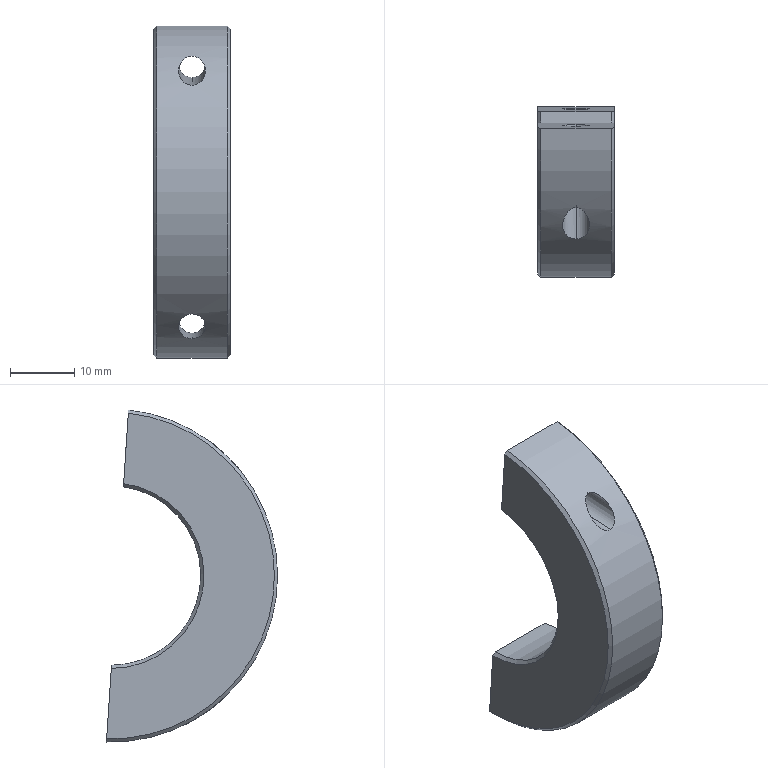Component | SolidWorks | TC020.05-08-1 | 1 solid | 14 faces | box 12 x 26.73 x 51.86 mm | volume 8299 mm3 | cylinder 6 | plane 4 | cone 4 | commonest cylinder face diameters 4.2 x4 28 x1 52 x1 | material Q235A
build123d program:
from build123d import *

# Parameters (mm, degrees)
SKETCH1_W          = 12
SKETCH1_H          = 12
SKETCH2_W          = 52
SKETCH2_H          = 2
CUT_EXTRUDE1_DEPTH = 39.678
M5_TAPPED_HOLE1_D  = 4.2
CHAMFER1_SIZE      = 0.5


with BuildPart() as part:
    # Sketch1 → Revolve1 (revolve)
    with BuildSketch(Plane.XY, mode=Mode.PRIVATE) as revolve1_sk:
        with Locations((0, 20)):
            Rectangle(SKETCH1_W, SKETCH1_H)
    revolve(revolve1_sk.sketch.rotate(Axis((0, 0, 0), (1, 0, 0)), 90), axis=Axis((0, 0, 0), (1, 0, 0)))

    # Sketch2 → Cut-Extrude1 (cut, through all)
    with BuildSketch(Plane(origin=(6, 0, 0), x_dir=(0, 0, -1), z_dir=(1, 0, 0))):
        Rectangle(SKETCH2_W, SKETCH2_H)
    extrude(amount=-CUT_EXTRUDE1_DEPTH, mode=Mode.SUBTRACT)


with BuildPart() as cut_extrude1_kept_piece:
    # of the separate pieces the step leaves, the one the design keeps (cut_extrude1_pieces_kept)
    add(part.part.solids().sort_by_distance((-6, 1, -13.964))[0])

    # M5 Tapped Hole1 (through all)
    with Locations(Plane.XZ.offset(-1)):
        with Locations((0, 20), (0, -20)):
            Hole(M5_TAPPED_HOLE1_D / 2)

    # Chamfer1
    chamfer1_edges = [cut_extrude1_kept_piece.edges().sort_by_distance(p)[0] for p in [
        (6, 26, 0),
        (-6, 26, 0),
        (-6, 14, 0),
        (6, 14, 0),
    ]]
    chamfer(chamfer1_edges, length=CHAMFER1_SIZE)


solid = cut_extrude1_kept_piece.part

# Placed as in the assembly
solid = solid.moved(Location((239.493, 30, 0), (3.804, 0, -180)))
STEP:
#1=COLOUR_RGB('',0.7922,0.8196,0.9333);
#2=FILL_AREA_STYLE_COLOUR('',#1);
#3=FILL_AREA_STYLE('',(#2));
#4=SURFACE_STYLE_FILL_AREA(#3);
#5=SURFACE_SIDE_STYLE('',(#4));
#6=SURFACE_STYLE_USAGE(.BOTH.,#5);
#7=PRESENTATION_STYLE_ASSIGNMENT((#6));
#8=CARTESIAN_POINT('',(9.429,0.7008,-0.9039));
#9=VERTEX_POINT('',#8);
#10=CARTESIAN_POINT('',(9.429,0.4871,-0.7524));
#11=VERTEX_POINT('',#10);
#12=CARTESIAN_POINT('',(9.429,0.7008,-0.9039));
#13=CARTESIAN_POINT('',(9.425,0.7008,-0.9039));
#14=CARTESIAN_POINT('',(9.422,0.7004,-0.9037));
#15=CARTESIAN_POINT('',(9.415,0.6989,-0.9029));
#16=CARTESIAN_POINT('',(9.411,0.6978,-0.9023));
#17=CARTESIAN_POINT('',(9.402,0.6937,-0.9001));
#18=CARTESIAN_POINT('',(9.396,0.6899,-0.8981));
#19=CARTESIAN_POINT('',(9.386,0.6813,-0.8933));
#20=CARTESIAN_POINT('',(9.381,0.6765,-0.8906));
#21=CARTESIAN_POINT('',(9.373,0.6663,-0.8848));
#22=CARTESIAN_POINT('',(9.37,0.6611,-0.8817));
#23=CARTESIAN_POINT('',(9.36,0.6448,-0.872));
#24=CARTESIAN_POINT('',(9.355,0.6333,-0.8648));
#25=CARTESIAN_POINT('',(9.349,0.6103,-0.8498));
#26=CARTESIAN_POINT('',(9.347,0.5988,-0.842));
#27=CARTESIAN_POINT('',(9.346,0.5816,-0.8297));
#28=CARTESIAN_POINT('',(9.346,0.5758,-0.8255));
#29=CARTESIAN_POINT('',(9.347,0.5645,-0.8171));
#30=CARTESIAN_POINT('',(9.348,0.5589,-0.8129));
#31=CARTESIAN_POINT('',(9.352,0.5425,-0.8001));
#32=CARTESIAN_POINT('',(9.356,0.5318,-0.7915));
#33=CARTESIAN_POINT('',(9.369,0.5126,-0.7753));
#34=CARTESIAN_POINT('',(9.378,0.5039,-0.7676));
#35=CARTESIAN_POINT('',(9.395,0.4942,-0.759));
#36=CARTESIAN_POINT('',(9.401,0.4916,-0.7566));
#37=CARTESIAN_POINT('',(9.411,0.4889,-0.7541));
#38=CARTESIAN_POINT('',(9.415,0.4883,-0.7535));
#39=CARTESIAN_POINT('',(9.422,0.4873,-0.7526));
#40=CARTESIAN_POINT('',(9.425,0.4871,-0.7524));
#41=CARTESIAN_POINT('',(9.429,0.4871,-0.7524));
#42=B_SPLINE_CURVE_WITH_KNOTS('',3,(#12,#13,#14,#15,#16,#17,#18,#19,#20,#21,#22,#23,#24,#25,#26,#27,#28,#29,#30,#31,#32,#33,#34,#35,#36,#37,#38,#39,#40,#41),.UNSPECIFIED.,.F.,.F.,(4,2,2,2,2,2,2,2,2,2,2,2,2,2,4),(0.008626,0.008896,0.009166,0.009706,0.01025,0.01079,0.01187,0.01295,0.01349,0.01403,0.01511,0.01619,0.01673,0.017,0.01727),.UNSPECIFIED.);
#43=EDGE_CURVE('',#9,#11,#42,.T.);
#44=ORIENTED_EDGE('',*,*,#43,.F.);
#45=CARTESIAN_POINT('',(9.429,1.2,-0.8708));
#46=VERTEX_POINT('',#45);
#47=CARTESIAN_POINT('',(9.429,1.2,-0.8708));
#48=DIRECTION('',(0.,0.9978,0.06635));
#49=VECTOR('',#48,39.37);
#50=LINE('',#47,#49);
#51=EDGE_CURVE('',#9,#46,#50,.T.);
#52=ORIENTED_EDGE('',*,*,#51,.T.);
#53=CARTESIAN_POINT('',(9.429,1.189,-0.7058));
#54=VERTEX_POINT('',#53);
#55=CARTESIAN_POINT('',(9.429,1.194,-0.7883));
#56=DIRECTION('',(0.,0.9978,0.06635));
#57=DIRECTION('',(0.,-0.06635,0.9978));
#58=AXIS2_PLACEMENT_3D('',#55,#56,#57);
#59=CIRCLE('',#58,0.08268);
#60=EDGE_CURVE('',#46,#54,#59,.T.);
#61=ORIENTED_EDGE('',*,*,#60,.T.);
#62=CARTESIAN_POINT('',(9.429,1.189,-0.7058));
#63=DIRECTION('',(0.,0.9978,0.06635));
#64=VECTOR('',#63,39.37);
#65=LINE('',#62,#64);
#66=EDGE_CURVE('',#11,#54,#65,.T.);
#67=ORIENTED_EDGE('',*,*,#66,.F.);
#68=EDGE_LOOP('',(#44,#52,#61,#67));
#69=FACE_OUTER_BOUND('',#68,.T.);
#70=CARTESIAN_POINT('',(9.429,1.194,-0.7883));
#71=DIRECTION('',(0.,0.9978,0.06635));
#72=DIRECTION('',(0.,-0.06635,0.9978));
#73=AXIS2_PLACEMENT_3D('',#70,#71,#72);
#74=CYLINDRICAL_SURFACE('',#73,0.08268);
#75=ADVANCED_FACE('',(#69),#74,.F.);
#76=CARTESIAN_POINT('',(9.429,0.3936,0.6539));
#77=VERTEX_POINT('',#76);
#78=CARTESIAN_POINT('',(9.429,0.5853,0.8324));
#79=VERTEX_POINT('',#78);
#80=CARTESIAN_POINT('',(9.429,0.3936,0.6539));
#81=CARTESIAN_POINT('',(9.422,0.3936,0.6539));
#82=CARTESIAN_POINT('',(9.415,0.3944,0.6549));
#83=CARTESIAN_POINT('',(9.401,0.3975,0.6586));
#84=CARTESIAN_POINT('',(9.395,0.3998,0.6613));
#85=CARTESIAN_POINT('',(9.384,0.4054,0.6679));
#86=CARTESIAN_POINT('',(9.379,0.4087,0.6718));
#87=CARTESIAN_POINT('',(9.37,0.416,0.6801));
#88=CARTESIAN_POINT('',(9.366,0.4201,0.6846));
#89=CARTESIAN_POINT('',(9.356,0.4328,0.6986));
#90=CARTESIAN_POINT('',(9.352,0.4421,0.7084));
#91=CARTESIAN_POINT('',(9.347,0.4617,0.7284));
#92=CARTESIAN_POINT('',(9.346,0.4718,0.7382));
#93=CARTESIAN_POINT('',(9.347,0.4923,0.7574));
#94=CARTESIAN_POINT('',(9.349,0.5029,0.7669));
#95=CARTESIAN_POINT('',(9.356,0.5236,0.7847));
#96=CARTESIAN_POINT('',(9.36,0.5339,0.7932));
#97=CARTESIAN_POINT('',(9.37,0.5489,0.8051));
#98=CARTESIAN_POINT('',(9.373,0.5538,0.8089));
#99=CARTESIAN_POINT('',(9.381,0.563,0.816));
#100=CARTESIAN_POINT('',(9.386,0.5675,0.8193));
#101=CARTESIAN_POINT('',(9.396,0.5753,0.8251));
#102=CARTESIAN_POINT('',(9.402,0.5788,0.8277));
#103=CARTESIAN_POINT('',(9.415,0.5838,0.8313));
#104=CARTESIAN_POINT('',(9.422,0.5853,0.8324));
#105=CARTESIAN_POINT('',(9.429,0.5853,0.8324));
#106=B_SPLINE_CURVE_WITH_KNOTS('',3,(#80,#81,#82,#83,#84,#85,#86,#87,#88,#89,#90,#91,#92,#93,#94,#95,#96,#97,#98,#99,#100,#101,#102,#103,#104,#105),.UNSPECIFIED.,.F.,.F.,(4,2,2,2,2,2,2,2,2,2,2,2,4),(0.008659,0.0092,0.009741,0.01028,0.01082,0.0119,0.01299,0.01407,0.01515,0.01569,0.01623,0.01677,0.01731),.UNSPECIFIED.);
#107=EDGE_CURVE('',#77,#79,#106,.T.);
#108=ORIENTED_EDGE('',*,*,#107,.F.);
#109=CARTESIAN_POINT('',(9.429,1.095,0.7006));
#110=VERTEX_POINT('',#109);
#111=CARTESIAN_POINT('',(9.429,1.095,0.7006));
#112=DIRECTION('',(0.,0.9978,0.06635));
#113=VECTOR('',#112,39.37);
#114=LINE('',#111,#113);
#115=EDGE_CURVE('',#77,#110,#114,.T.);
#116=ORIENTED_EDGE('',*,*,#115,.T.);
#117=CARTESIAN_POINT('',(9.429,1.084,0.8655));
#118=VERTEX_POINT('',#117);
#119=CARTESIAN_POINT('',(9.429,1.09,0.7831));
#120=DIRECTION('',(0.,0.9978,0.06635));
#121=DIRECTION('',(0.,-0.06635,0.9978));
#122=AXIS2_PLACEMENT_3D('',#119,#120,#121);
#123=CIRCLE('',#122,0.08268);
#124=EDGE_CURVE('',#110,#118,#123,.T.);
#125=ORIENTED_EDGE('',*,*,#124,.T.);
#126=CARTESIAN_POINT('',(9.429,1.084,0.8655));
#127=DIRECTION('',(0.,0.9978,0.06635));
#128=VECTOR('',#127,39.37);
#129=LINE('',#126,#128);
#130=EDGE_CURVE('',#79,#118,#129,.T.);
#131=ORIENTED_EDGE('',*,*,#130,.F.);
#132=EDGE_LOOP('',(#108,#116,#125,#131));
#133=FACE_OUTER_BOUND('',#132,.T.);
#134=CARTESIAN_POINT('',(9.429,1.09,0.7831));
#135=DIRECTION('',(0.,0.9978,0.06635));
#136=DIRECTION('',(0.,-0.06635,0.9978));
#137=AXIS2_PLACEMENT_3D('',#134,#135,#136);
#138=CYLINDRICAL_SURFACE('',#137,0.08268);
#139=ADVANCED_FACE('',(#133),#138,.F.);
#140=CARTESIAN_POINT('',(9.645,1.178,-0.5512));
#141=VERTEX_POINT('',#140);
#142=CARTESIAN_POINT('',(9.212,1.178,-0.5512));
#143=VERTEX_POINT('',#142);
#144=CARTESIAN_POINT('',(9.429,1.178,-0.5512));
#145=DIRECTION('',(-1.,0.,0.));
#146=VECTOR('',#145,39.37);
#147=LINE('',#144,#146);
#148=EDGE_CURVE('',#141,#143,#147,.T.);
#149=ORIENTED_EDGE('',*,*,#148,.T.);
#150=CARTESIAN_POINT('',(9.212,1.105,0.5459));
#151=VERTEX_POINT('',#150);
#152=CARTESIAN_POINT('',(9.212,1.181,0.));
#153=DIRECTION('',(-1.,0.,0.));
#154=DIRECTION('',(0.,-0.06635,0.9978));
#155=AXIS2_PLACEMENT_3D('',#152,#153,#154);
#156=CIRCLE('',#155,0.5512);
#157=EDGE_CURVE('',#143,#151,#156,.T.);
#158=ORIENTED_EDGE('',*,*,#157,.T.);
#159=CARTESIAN_POINT('',(9.645,1.105,0.5459));
#160=VERTEX_POINT('',#159);
#161=CARTESIAN_POINT('',(9.429,1.105,0.5459));
#162=DIRECTION('',(1.,0.,0.));
#163=VECTOR('',#162,39.37);
#164=LINE('',#161,#163);
#165=EDGE_CURVE('',#151,#160,#164,.T.);
#166=ORIENTED_EDGE('',*,*,#165,.T.);
#167=CARTESIAN_POINT('',(9.645,1.181,0.));
#168=DIRECTION('',(1.,0.,0.));
#169=DIRECTION('',(0.,0.06635,-0.9978));
#170=AXIS2_PLACEMENT_3D('',#167,#168,#169);
#171=CIRCLE('',#170,0.5512);
#172=EDGE_CURVE('',#160,#141,#171,.T.);
#173=ORIENTED_EDGE('',*,*,#172,.T.);
#174=EDGE_LOOP('',(#149,#158,#166,#173));
#175=FACE_OUTER_BOUND('',#174,.T.);
#176=CARTESIAN_POINT('',(9.429,1.181,0.));
#177=DIRECTION('',(-1.,0.,0.));
#178=DIRECTION('',(0.,0.06635,-0.9978));
#179=AXIS2_PLACEMENT_3D('',#176,#177,#178);
#180=CYLINDRICAL_SURFACE('',#179,0.5512);
#181=ADVANCED_FACE('',(#175),#180,.F.);
#182=CARTESIAN_POINT('',(9.665,1.18,-0.5709));
#183=VERTEX_POINT('',#182);
#184=CARTESIAN_POINT('',(9.665,1.208,-1.004));
#185=VERTEX_POINT('',#184);
#186=CARTESIAN_POINT('',(9.665,1.21,-1.024));
#187=DIRECTION('',(0.,0.06635,-0.9978));
#188=VECTOR('',#187,39.37);
#189=LINE('',#186,#188);
#190=EDGE_CURVE('',#183,#185,#189,.T.);
#191=ORIENTED_EDGE('',*,*,#190,.F.);
#192=CARTESIAN_POINT('',(9.665,1.104,0.5656));
#193=VERTEX_POINT('',#192);
#194=CARTESIAN_POINT('',(9.665,1.181,0.));
#195=DIRECTION('',(-1.,0.,0.));
#196=DIRECTION('',(0.,0.06635,-0.9978));
#197=AXIS2_PLACEMENT_3D('',#194,#195,#196);
#198=CIRCLE('',#197,0.5709);
#199=EDGE_CURVE('',#183,#193,#198,.T.);
#200=ORIENTED_EDGE('',*,*,#199,.T.);
#201=CARTESIAN_POINT('',(9.665,1.075,0.9983));
#202=VERTEX_POINT('',#201);
#203=CARTESIAN_POINT('',(9.665,1.21,-1.024));
#204=DIRECTION('',(0.,0.06635,-0.9978));
#205=VECTOR('',#204,39.37);
#206=LINE('',#203,#205);
#207=EDGE_CURVE('',#202,#193,#206,.T.);
#208=ORIENTED_EDGE('',*,*,#207,.F.);
#209=CARTESIAN_POINT('',(9.665,1.181,0.));
#210=DIRECTION('',(1.,0.,0.));
#211=DIRECTION('',(0.,0.06635,-0.9978));
#212=AXIS2_PLACEMENT_3D('',#209,#210,#211);
#213=CIRCLE('',#212,1.004);
#214=EDGE_CURVE('',#202,#185,#213,.T.);
#215=ORIENTED_EDGE('',*,*,#214,.T.);
#216=EDGE_LOOP('',(#191,#200,#208,#215));
#217=FACE_OUTER_BOUND('',#216,.T.);
#218=CARTESIAN_POINT('',(9.665,0.6311,-0.03657));
#219=DIRECTION('',(-1.,0.,0.));
#220=DIRECTION('',(0.,0.06635,-0.9978));
#221=AXIS2_PLACEMENT_3D('',#218,#219,#220);
#222=PLANE('',#221);
#223=ADVANCED_FACE('',(#217),#222,.F.);
#224=CARTESIAN_POINT('',(9.429,0.4871,-0.7524));
#225=CARTESIAN_POINT('',(9.436,0.4871,-0.7524));
#226=CARTESIAN_POINT('',(9.443,0.488,-0.7533));
#227=CARTESIAN_POINT('',(9.456,0.4916,-0.7566));
#228=CARTESIAN_POINT('',(9.463,0.4942,-0.7589));
#229=CARTESIAN_POINT('',(9.474,0.5007,-0.7647));
#230=CARTESIAN_POINT('',(9.479,0.5044,-0.7681));
#231=CARTESIAN_POINT('',(9.488,0.5128,-0.7753));
#232=CARTESIAN_POINT('',(9.492,0.5174,-0.7793));
#233=CARTESIAN_POINT('',(9.498,0.527,-0.7874));
#234=CARTESIAN_POINT('',(9.501,0.532,-0.7916));
#235=CARTESIAN_POINT('',(9.505,0.5425,-0.8));
#236=CARTESIAN_POINT('',(9.507,0.5479,-0.8043));
#237=CARTESIAN_POINT('',(9.511,0.5644,-0.8171));
#238=CARTESIAN_POINT('',(9.512,0.5757,-0.8255));
#239=CARTESIAN_POINT('',(9.511,0.5987,-0.8419));
#240=CARTESIAN_POINT('',(9.509,0.6104,-0.8499));
#241=CARTESIAN_POINT('',(9.502,0.6333,-0.8648));
#242=CARTESIAN_POINT('',(9.497,0.6448,-0.872));
#243=CARTESIAN_POINT('',(9.488,0.6611,-0.8817));
#244=CARTESIAN_POINT('',(9.485,0.6664,-0.8848));
#245=CARTESIAN_POINT('',(9.476,0.6765,-0.8906));
#246=CARTESIAN_POINT('',(9.472,0.6813,-0.8933));
#247=CARTESIAN_POINT('',(9.462,0.6899,-0.8981));
#248=CARTESIAN_POINT('',(9.456,0.6937,-0.9001));
#249=CARTESIAN_POINT('',(9.443,0.6992,-0.9031));
#250=CARTESIAN_POINT('',(9.436,0.7008,-0.9039));
#251=CARTESIAN_POINT('',(9.429,0.7008,-0.9039));
#252=B_SPLINE_CURVE_WITH_KNOTS('',3,(#224,#225,#226,#227,#228,#229,#230,#231,#232,#233,#234,#235,#236,#237,#238,#239,#240,#241,#242,#243,#244,#245,#246,#247,#248,#249,#250,#251),.UNSPECIFIED.,.F.,.F.,(4,2,2,2,2,2,2,2,2,2,2,2,2,4),(0.,0.0005391,0.001078,0.001617,0.002156,0.002696,0.003235,0.004313,0.005391,0.006469,0.007008,0.007547,0.008087,0.008626),.UNSPECIFIED.);
#253=EDGE_CURVE('',#11,#9,#252,.T.);
#254=ORIENTED_EDGE('',*,*,#253,.T.);
#255=ORIENTED_EDGE('',*,*,#43,.T.);
#256=EDGE_LOOP('',(#254,#255));
#257=FACE_BOUND('',#256,.T.);
#258=CARTESIAN_POINT('',(9.429,0.5853,0.8324));
#259=CARTESIAN_POINT('',(9.432,0.5853,0.8324));
#260=CARTESIAN_POINT('',(9.436,0.585,0.8321));
#261=CARTESIAN_POINT('',(9.443,0.5836,0.8311));
#262=CARTESIAN_POINT('',(9.446,0.5826,0.8304));
#263=CARTESIAN_POINT('',(9.456,0.5788,0.8277));
#264=CARTESIAN_POINT('',(9.462,0.5753,0.8251));
#265=CARTESIAN_POINT('',(9.477,0.5635,0.8164));
#266=CARTESIAN_POINT('',(9.485,0.5538,0.809));
#267=CARTESIAN_POINT('',(9.494,0.539,0.7972));
#268=CARTESIAN_POINT('',(9.497,0.5339,0.7931));
#269=CARTESIAN_POINT('',(9.502,0.5237,0.7846));
#270=CARTESIAN_POINT('',(9.504,0.5184,0.7802));
#271=CARTESIAN_POINT('',(9.509,0.5028,0.7667));
#272=CARTESIAN_POINT('',(9.511,0.4924,0.7575));
#273=CARTESIAN_POINT('',(9.512,0.4719,0.7382));
#274=CARTESIAN_POINT('',(9.511,0.4616,0.7282));
#275=CARTESIAN_POINT('',(9.507,0.447,0.7134));
#276=CARTESIAN_POINT('',(9.505,0.4423,0.7085));
#277=CARTESIAN_POINT('',(9.501,0.433,0.6987));
#278=CARTESIAN_POINT('',(9.498,0.4285,0.6938));
#279=CARTESIAN_POINT('',(9.489,0.4158,0.6799));
#280=CARTESIAN_POINT('',(9.48,0.4082,0.6712));
#281=CARTESIAN_POINT('',(9.463,0.3998,0.6613));
#282=CARTESIAN_POINT('',(9.456,0.3975,0.6586));
#283=CARTESIAN_POINT('',(9.446,0.3952,0.6558));
#284=CARTESIAN_POINT('',(9.443,0.3946,0.6551));
#285=CARTESIAN_POINT('',(9.436,0.3938,0.6542));
#286=CARTESIAN_POINT('',(9.432,0.3936,0.6539));
#287=CARTESIAN_POINT('',(9.429,0.3936,0.6539));
#288=B_SPLINE_CURVE_WITH_KNOTS('',3,(#258,#259,#260,#261,#262,#263,#264,#265,#266,#267,#268,#269,#270,#271,#272,#273,#274,#275,#276,#277,#278,#279,#280,#281,#282,#283,#284,#285,#286,#287),.UNSPECIFIED.,.F.,.F.,(4,2,2,2,2,2,2,2,2,2,2,2,2,2,4),(0.,0.0002706,0.0005412,0.001082,0.002165,0.002706,0.003247,0.004329,0.005412,0.005953,0.006494,0.007577,0.008118,0.008388,0.008659),.UNSPECIFIED.);
#289=EDGE_CURVE('',#79,#77,#288,.T.);
#290=ORIENTED_EDGE('',*,*,#289,.T.);
#291=ORIENTED_EDGE('',*,*,#107,.T.);
#292=EDGE_LOOP('',(#290,#291));
#293=FACE_BOUND('',#292,.T.);
#294=CARTESIAN_POINT('',(9.645,1.074,1.018));
#295=VERTEX_POINT('',#294);
#296=CARTESIAN_POINT('',(9.212,1.074,1.018));
#297=VERTEX_POINT('',#296);
#298=CARTESIAN_POINT('',(9.429,1.074,1.018));
#299=DIRECTION('',(-1.,0.,0.));
#300=VECTOR('',#299,39.37);
#301=LINE('',#298,#300);
#302=EDGE_CURVE('',#295,#297,#301,.T.);
#303=ORIENTED_EDGE('',*,*,#302,.T.);
#304=CARTESIAN_POINT('',(9.212,1.21,-1.023));
#305=VERTEX_POINT('',#304);
#306=CARTESIAN_POINT('',(9.212,1.181,0.));
#307=DIRECTION('',(1.,0.,0.));
#308=DIRECTION('',(0.,-0.06635,0.9978));
#309=AXIS2_PLACEMENT_3D('',#306,#307,#308);
#310=CIRCLE('',#309,1.024);
#311=EDGE_CURVE('',#297,#305,#310,.T.);
#312=ORIENTED_EDGE('',*,*,#311,.T.);
#313=CARTESIAN_POINT('',(9.645,1.21,-1.023));
#314=VERTEX_POINT('',#313);
#315=CARTESIAN_POINT('',(9.429,1.21,-1.023));
#316=DIRECTION('',(1.,0.,0.));
#317=VECTOR('',#316,39.37);
#318=LINE('',#315,#317);
#319=EDGE_CURVE('',#305,#314,#318,.T.);
#320=ORIENTED_EDGE('',*,*,#319,.T.);
#321=CARTESIAN_POINT('',(9.645,1.181,0.));
#322=DIRECTION('',(-1.,0.,0.));
#323=DIRECTION('',(0.,0.06635,-0.9978));
#324=AXIS2_PLACEMENT_3D('',#321,#322,#323);
#325=CIRCLE('',#324,1.024);
#326=EDGE_CURVE('',#314,#295,#325,.T.);
#327=ORIENTED_EDGE('',*,*,#326,.T.);
#328=EDGE_LOOP('',(#303,#312,#320,#327));
#329=FACE_OUTER_BOUND('',#328,.T.);
#330=CARTESIAN_POINT('',(9.429,1.181,0.));
#331=DIRECTION('',(-1.,0.,0.));
#332=DIRECTION('',(0.,0.06635,-0.9978));
#333=AXIS2_PLACEMENT_3D('',#330,#331,#332);
#334=CYLINDRICAL_SURFACE('',#333,1.024);
#335=ADVANCED_FACE('',(#257,#293,#329),#334,.T.);
#336=CARTESIAN_POINT('',(9.193,1.075,0.9983));
#337=VERTEX_POINT('',#336);
#338=CARTESIAN_POINT('',(9.193,1.104,0.5656));
#339=VERTEX_POINT('',#338);
#340=CARTESIAN_POINT('',(9.193,1.21,-1.024));
#341=DIRECTION('',(0.,0.06635,-0.9978));
#342=VECTOR('',#341,39.37);
#343=LINE('',#340,#342);
#344=EDGE_CURVE('',#337,#339,#343,.T.);
#345=ORIENTED_EDGE('',*,*,#344,.T.);
#346=CARTESIAN_POINT('',(9.193,1.18,-0.5709));
#347=VERTEX_POINT('',#346);
#348=CARTESIAN_POINT('',(9.193,1.181,0.));
#349=DIRECTION('',(1.,0.,0.));
#350=DIRECTION('',(0.,-0.06635,0.9978));
#351=AXIS2_PLACEMENT_3D('',#348,#349,#350);
#352=CIRCLE('',#351,0.5709);
#353=EDGE_CURVE('',#339,#347,#352,.T.);
#354=ORIENTED_EDGE('',*,*,#353,.T.);
#355=CARTESIAN_POINT('',(9.193,1.208,-1.004));
#356=VERTEX_POINT('',#355);
#357=CARTESIAN_POINT('',(9.193,1.21,-1.024));
#358=DIRECTION('',(0.,0.06635,-0.9978));
#359=VECTOR('',#358,39.37);
#360=LINE('',#357,#359);
#361=EDGE_CURVE('',#347,#356,#360,.T.);
#362=ORIENTED_EDGE('',*,*,#361,.T.);
#363=CARTESIAN_POINT('',(9.193,1.181,0.));
#364=DIRECTION('',(-1.,0.,0.));
#365=DIRECTION('',(0.,-0.06635,0.9978));
#366=AXIS2_PLACEMENT_3D('',#363,#364,#365);
#367=CIRCLE('',#366,1.004);
#368=EDGE_CURVE('',#356,#337,#367,.T.);
#369=ORIENTED_EDGE('',*,*,#368,.T.);
#370=EDGE_LOOP('',(#345,#354,#362,#369));
#371=FACE_OUTER_BOUND('',#370,.T.);
#372=CARTESIAN_POINT('',(9.193,0.6311,-0.03657));
#373=DIRECTION('',(1.,0.,0.));
#374=DIRECTION('',(0.,-0.06635,0.9978));
#375=AXIS2_PLACEMENT_3D('',#372,#373,#374);
#376=PLANE('',#375);
#377=ADVANCED_FACE('',(#371),#376,.F.);
#378=CARTESIAN_POINT('',(9.429,1.194,-0.7883));
#379=DIRECTION('',(0.,0.9978,0.06635));
#380=DIRECTION('',(0.,-0.06635,0.9978));
#381=AXIS2_PLACEMENT_3D('',#378,#379,#380);
#382=CIRCLE('',#381,0.08268);
#383=EDGE_CURVE('',#54,#46,#382,.T.);
#384=ORIENTED_EDGE('',*,*,#383,.F.);
#385=ORIENTED_EDGE('',*,*,#60,.F.);
#386=EDGE_LOOP('',(#384,#385));
#387=FACE_BOUND('',#386,.T.);
#388=ORIENTED_EDGE('',*,*,#361,.F.);
#389=CARTESIAN_POINT('',(9.193,1.18,-0.5709));
#390=CARTESIAN_POINT('',(9.199,1.179,-0.5643));
#391=CARTESIAN_POINT('',(9.206,1.179,-0.5577));
#392=CARTESIAN_POINT('',(9.212,1.178,-0.5512));
#393=B_SPLINE_CURVE_WITH_KNOTS('',3,(#389,#390,#391,#392),.UNSPECIFIED.,.F.,.F.,(4,4),(0.,0.000708),.UNSPECIFIED.);
#394=EDGE_CURVE('',#347,#143,#393,.T.);
#395=ORIENTED_EDGE('',*,*,#394,.T.);
#396=ORIENTED_EDGE('',*,*,#148,.F.);
#397=CARTESIAN_POINT('',(9.645,1.178,-0.5512));
#398=CARTESIAN_POINT('',(9.652,1.179,-0.5577));
#399=CARTESIAN_POINT('',(9.659,1.179,-0.5643));
#400=CARTESIAN_POINT('',(9.665,1.18,-0.5709));
#401=B_SPLINE_CURVE_WITH_KNOTS('',3,(#397,#398,#399,#400),.UNSPECIFIED.,.F.,.F.,(4,4),(0.,0.000708),.UNSPECIFIED.);
#402=EDGE_CURVE('',#141,#183,#401,.T.);
#403=ORIENTED_EDGE('',*,*,#402,.T.);
#404=ORIENTED_EDGE('',*,*,#190,.T.);
#405=CARTESIAN_POINT('',(9.665,1.208,-1.004));
#406=CARTESIAN_POINT('',(9.659,1.209,-1.01));
#407=CARTESIAN_POINT('',(9.652,1.209,-1.017));
#408=CARTESIAN_POINT('',(9.645,1.21,-1.023));
#409=B_SPLINE_CURVE_WITH_KNOTS('',3,(#405,#406,#407,#408),.UNSPECIFIED.,.F.,.F.,(4,4),(0.,0.0007074),.UNSPECIFIED.);
#410=EDGE_CURVE('',#185,#314,#409,.T.);
#411=ORIENTED_EDGE('',*,*,#410,.T.);
#412=ORIENTED_EDGE('',*,*,#319,.F.);
#413=CARTESIAN_POINT('',(9.212,1.21,-1.023));
#414=CARTESIAN_POINT('',(9.206,1.209,-1.017));
#415=CARTESIAN_POINT('',(9.199,1.209,-1.01));
#416=CARTESIAN_POINT('',(9.193,1.208,-1.004));
#417=B_SPLINE_CURVE_WITH_KNOTS('',3,(#413,#414,#415,#416),.UNSPECIFIED.,.F.,.F.,(4,4),(0.,0.0007074),.UNSPECIFIED.);
#418=EDGE_CURVE('',#305,#356,#417,.T.);
#419=ORIENTED_EDGE('',*,*,#418,.T.);
#420=EDGE_LOOP('',(#388,#395,#396,#403,#404,#411,#412,#419));
#421=FACE_OUTER_BOUND('',#420,.T.);
#422=CARTESIAN_POINT('',(9.193,1.21,-1.024));
#423=DIRECTION('',(0.,-0.9978,-0.06635));
#424=DIRECTION('',(0.,0.06635,-0.9978));
#425=AXIS2_PLACEMENT_3D('',#422,#423,#424);
#426=PLANE('',#425);
#427=ADVANCED_FACE('',(#387,#421),#426,.F.);
#428=CARTESIAN_POINT('',(9.429,1.09,0.7831));
#429=DIRECTION('',(0.,0.9978,0.06635));
#430=DIRECTION('',(0.,-0.06635,0.9978));
#431=AXIS2_PLACEMENT_3D('',#428,#429,#430);
#432=CIRCLE('',#431,0.08268);
#433=EDGE_CURVE('',#118,#110,#432,.T.);
#434=ORIENTED_EDGE('',*,*,#433,.F.);
#435=ORIENTED_EDGE('',*,*,#124,.F.);
#436=EDGE_LOOP('',(#434,#435));
#437=FACE_BOUND('',#436,.T.);
#438=ORIENTED_EDGE('',*,*,#165,.F.);
#439=CARTESIAN_POINT('',(9.212,1.105,0.5459));
#440=CARTESIAN_POINT('',(9.206,1.105,0.5525));
#441=CARTESIAN_POINT('',(9.199,1.104,0.5591));
#442=CARTESIAN_POINT('',(9.193,1.104,0.5656));
#443=B_SPLINE_CURVE_WITH_KNOTS('',3,(#439,#440,#441,#442),.UNSPECIFIED.,.F.,.F.,(4,4),(0.,0.000708),.UNSPECIFIED.);
#444=EDGE_CURVE('',#151,#339,#443,.T.);
#445=ORIENTED_EDGE('',*,*,#444,.T.);
#446=ORIENTED_EDGE('',*,*,#344,.F.);
#447=CARTESIAN_POINT('',(9.193,1.075,0.9983));
#448=CARTESIAN_POINT('',(9.199,1.075,1.005));
#449=CARTESIAN_POINT('',(9.206,1.074,1.011));
#450=CARTESIAN_POINT('',(9.212,1.074,1.018));
#451=B_SPLINE_CURVE_WITH_KNOTS('',3,(#447,#448,#449,#450),.UNSPECIFIED.,.F.,.F.,(4,4),(0.,0.0007074),.UNSPECIFIED.);
#452=EDGE_CURVE('',#337,#297,#451,.T.);
#453=ORIENTED_EDGE('',*,*,#452,.T.);
#454=ORIENTED_EDGE('',*,*,#302,.F.);
#455=CARTESIAN_POINT('',(9.645,1.074,1.018));
#456=CARTESIAN_POINT('',(9.652,1.074,1.011));
#457=CARTESIAN_POINT('',(9.659,1.075,1.005));
#458=CARTESIAN_POINT('',(9.665,1.075,0.9983));
#459=B_SPLINE_CURVE_WITH_KNOTS('',3,(#455,#456,#457,#458),.UNSPECIFIED.,.F.,.F.,(4,4),(0.,0.0007074),.UNSPECIFIED.);
#460=EDGE_CURVE('',#295,#202,#459,.T.);
#461=ORIENTED_EDGE('',*,*,#460,.T.);
#462=ORIENTED_EDGE('',*,*,#207,.T.);
#463=CARTESIAN_POINT('',(9.665,1.104,0.5656));
#464=CARTESIAN_POINT('',(9.659,1.104,0.5591));
#465=CARTESIAN_POINT('',(9.652,1.105,0.5525));
#466=CARTESIAN_POINT('',(9.645,1.105,0.5459));
#467=B_SPLINE_CURVE_WITH_KNOTS('',3,(#463,#464,#465,#466),.UNSPECIFIED.,.F.,.F.,(4,4),(0.,0.000708),.UNSPECIFIED.);
#468=EDGE_CURVE('',#193,#160,#467,.T.);
#469=ORIENTED_EDGE('',*,*,#468,.T.);
#470=EDGE_LOOP('',(#438,#445,#446,#453,#454,#461,#462,#469));
#471=FACE_OUTER_BOUND('',#470,.T.);
#472=CARTESIAN_POINT('',(9.193,1.21,-1.024));
#473=DIRECTION('',(0.,-0.9978,-0.06635));
#474=DIRECTION('',(0.,0.06635,-0.9978));
#475=AXIS2_PLACEMENT_3D('',#472,#473,#474);
#476=PLANE('',#475);
#477=ADVANCED_FACE('',(#437,#471),#476,.F.);
#478=ORIENTED_EDGE('',*,*,#115,.F.);
#479=ORIENTED_EDGE('',*,*,#289,.F.);
#480=ORIENTED_EDGE('',*,*,#130,.T.);
#481=ORIENTED_EDGE('',*,*,#433,.T.);
#482=EDGE_LOOP('',(#478,#479,#480,#481));
#483=FACE_OUTER_BOUND('',#482,.T.);
#484=CARTESIAN_POINT('',(9.429,1.09,0.7831));
#485=DIRECTION('',(0.,0.9978,0.06635));
#486=DIRECTION('',(0.,-0.06635,0.9978));
#487=AXIS2_PLACEMENT_3D('',#484,#485,#486);
#488=CYLINDRICAL_SURFACE('',#487,0.08268);
#489=ADVANCED_FACE('',(#483),#488,.F.);
#490=ORIENTED_EDGE('',*,*,#51,.F.);
#491=ORIENTED_EDGE('',*,*,#253,.F.);
#492=ORIENTED_EDGE('',*,*,#66,.T.);
#493=ORIENTED_EDGE('',*,*,#383,.T.);
#494=EDGE_LOOP('',(#490,#491,#492,#493));
#495=FACE_OUTER_BOUND('',#494,.T.);
#496=CARTESIAN_POINT('',(9.429,1.194,-0.7883));
#497=DIRECTION('',(0.,0.9978,0.06635));
#498=DIRECTION('',(0.,-0.06635,0.9978));
#499=AXIS2_PLACEMENT_3D('',#496,#497,#498);
#500=CYLINDRICAL_SURFACE('',#499,0.08268);
#501=ADVANCED_FACE('',(#495),#500,.F.);
#502=ORIENTED_EDGE('',*,*,#394,.F.);
#503=ORIENTED_EDGE('',*,*,#353,.F.);
#504=ORIENTED_EDGE('',*,*,#444,.F.);
#505=ORIENTED_EDGE('',*,*,#157,.F.);
#506=EDGE_LOOP('',(#502,#503,#504,#505));
#507=FACE_OUTER_BOUND('',#506,.T.);
#508=CARTESIAN_POINT('',(9.212,1.181,0.));
#509=DIRECTION('',(-1.,0.,0.));
#510=DIRECTION('',(0.,0.06635,-0.9978));
#511=AXIS2_PLACEMENT_3D('',#508,#509,#510);
#512=CONICAL_SURFACE('',#511,0.5512,0.7854);
#513=ADVANCED_FACE('',(#507),#512,.F.);
#514=ORIENTED_EDGE('',*,*,#418,.F.);
#515=ORIENTED_EDGE('',*,*,#311,.F.);
#516=ORIENTED_EDGE('',*,*,#452,.F.);
#517=ORIENTED_EDGE('',*,*,#368,.F.);
#518=EDGE_LOOP('',(#514,#515,#516,#517));
#519=FACE_OUTER_BOUND('',#518,.T.);
#520=CARTESIAN_POINT('',(9.193,1.181,0.));
#521=DIRECTION('',(1.,0.,0.));
#522=DIRECTION('',(0.,-0.06635,0.9978));
#523=AXIS2_PLACEMENT_3D('',#520,#521,#522);
#524=CONICAL_SURFACE('',#523,1.004,0.7854);
#525=ADVANCED_FACE('',(#519),#524,.T.);
#526=ORIENTED_EDGE('',*,*,#402,.F.);
#527=ORIENTED_EDGE('',*,*,#172,.F.);
#528=ORIENTED_EDGE('',*,*,#468,.F.);
#529=ORIENTED_EDGE('',*,*,#199,.F.);
#530=EDGE_LOOP('',(#526,#527,#528,#529));
#531=FACE_OUTER_BOUND('',#530,.T.);
#532=CARTESIAN_POINT('',(9.665,1.181,0.));
#533=DIRECTION('',(1.,0.,0.));
#534=DIRECTION('',(0.,-0.06635,0.9978));
#535=AXIS2_PLACEMENT_3D('',#532,#533,#534);
#536=CONICAL_SURFACE('',#535,0.5709,0.7854);
#537=ADVANCED_FACE('',(#531),#536,.F.);
#538=ORIENTED_EDGE('',*,*,#410,.F.);
#539=ORIENTED_EDGE('',*,*,#214,.F.);
#540=ORIENTED_EDGE('',*,*,#460,.F.);
#541=ORIENTED_EDGE('',*,*,#326,.F.);
#542=EDGE_LOOP('',(#538,#539,#540,#541));
#543=FACE_OUTER_BOUND('',#542,.T.);
#544=CARTESIAN_POINT('',(9.645,1.181,0.));
#545=DIRECTION('',(-1.,0.,0.));
#546=DIRECTION('',(0.,0.06635,-0.9978));
#547=AXIS2_PLACEMENT_3D('',#544,#545,#546);
#548=CONICAL_SURFACE('',#547,1.024,0.7854);
#549=ADVANCED_FACE('',(#543),#548,.T.);
#550=CLOSED_SHELL('',(#75,#139,#181,#223,#335,#377,#427,#477,#489,#501,#513,#525,#537,#549));
#551=MANIFOLD_SOLID_BREP('',#550);
#552=STYLED_ITEM('',(#7),#551);
#553=PRESENTATION_LAYER_ASSIGNMENT('','',(#552));
#554=CARTESIAN_POINT('',(0.,0.,0.));
#555=DIRECTION('',(0.,0.,1.));
#556=DIRECTION('',(1.,0.,0.));
#557=AXIS2_PLACEMENT_3D('',#554,#555,#556);
#558=(LENGTH_UNIT()NAMED_UNIT(*)SI_UNIT($,.METRE.));
#559=LENGTH_MEASURE_WITH_UNIT(LENGTH_MEASURE(0.0254),#558);
#560=DIMENSIONAL_EXPONENTS(1.,0.,0.,0.,0.,0.,0.);
#561=(CONVERSION_BASED_UNIT('',#559)LENGTH_UNIT()NAMED_UNIT(#560));
#562=UNCERTAINTY_MEASURE_WITH_UNIT(LENGTH_MEASURE(0.00001),#561,'','');
#563=(NAMED_UNIT(*)PLANE_ANGLE_UNIT()SI_UNIT($,.RADIAN.));
#564=(NAMED_UNIT(*)SI_UNIT($,.STERADIAN.)SOLID_ANGLE_UNIT());
#565=(GEOMETRIC_REPRESENTATION_CONTEXT(3)GLOBAL_UNCERTAINTY_ASSIGNED_CONTEXT((#562))GLOBAL_UNIT_ASSIGNED_CONTEXT((#561,#563,#564))REPRESENTATION_CONTEXT('',''));
#566=ADVANCED_BREP_SHAPE_REPRESENTATION('',(#551,#557),#565);
#567=(LENGTH_UNIT()NAMED_UNIT(*)SI_UNIT($,.METRE.));
#568=LENGTH_MEASURE_WITH_UNIT(LENGTH_MEASURE(0.0254),#567);
#569=DIMENSIONAL_EXPONENTS(1.,0.,0.,0.,0.,0.,0.);
#570=(CONVERSION_BASED_UNIT('',#568)LENGTH_UNIT()NAMED_UNIT(#569));
#571=UNCERTAINTY_MEASURE_WITH_UNIT(LENGTH_MEASURE(0.00001),#570,'','');
#572=(NAMED_UNIT(*)PLANE_ANGLE_UNIT()SI_UNIT($,.RADIAN.));
#573=(NAMED_UNIT(*)SI_UNIT($,.STERADIAN.)SOLID_ANGLE_UNIT());
#574=(GEOMETRIC_REPRESENTATION_CONTEXT(3)GLOBAL_UNCERTAINTY_ASSIGNED_CONTEXT((#571))GLOBAL_UNIT_ASSIGNED_CONTEXT((#570,#572,#573))REPRESENTATION_CONTEXT('',''));
#575=MECHANICAL_DESIGN_GEOMETRIC_PRESENTATION_REPRESENTATION('',(#552),#574);